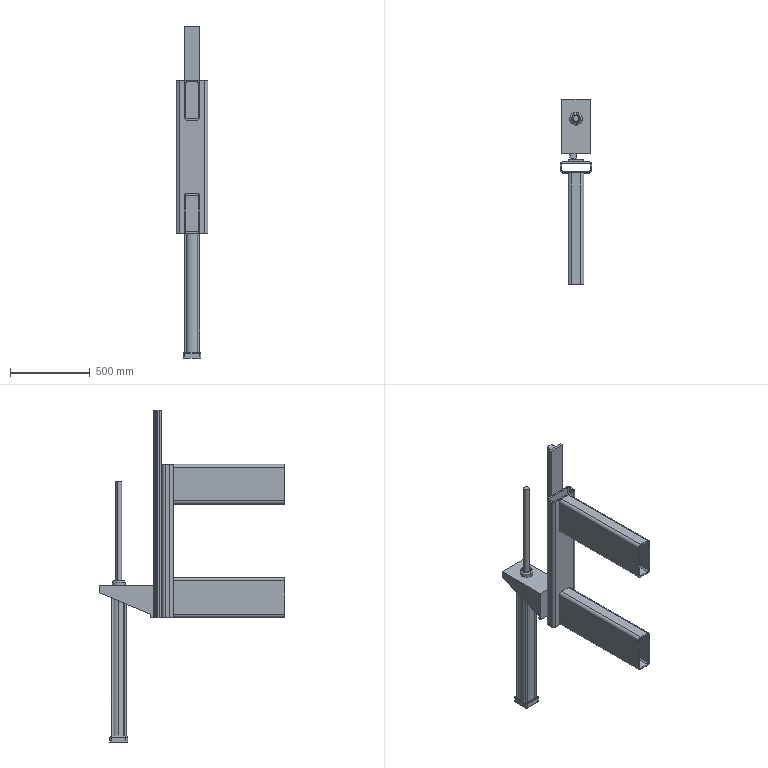Assembly | SolidWorks | mm | 15 component files | 15 solids | 255 faces | box 200 x 1164 x 2080 mm | volume 28088641 mm3 | cylinder 137 | plane 108 | torus 10 | commonest cylinder face diameters 30 x26 15.5 x26 15 x24 20 x20 40 x12 10 x11 85 x6 95 x4
Bill of materials:
CylinderBaseBaffle | 1 |  | Rectangular block with one sloped face. It is tall at one end and tapers to a thin end at the other. One round through-hole runs top to bottom, and a small step sits at the bottom of the tall end.
CylinderJoint | 1 | 1023 Carbon Steel Plate (SS) | Square flange base with rounded corners and edges, four corner through-holes, and a cylindrical boss in the middle. The boss has a rounded top edge and a central through-bore.
CylinderRod1 | 1 | 201 Annealed Stainless Steel (SS) | Solid round rod: a plain cylinder with flat ends.
CylinderWall1 | 1 | 201 Annealed Stainless Steel (SS) | Thin-walled round tube with open ends.
GuideRail2100 | 1 |  | Long, slender straight profile with a shaped cross-section and a row of evenly spaced small holes along one face.
GuideRailPad | 1 | Alloy Steel | Thin, flat rectangular strip or bar with no holes or other features.
MountingBracket | 1 | 1023 Carbon Steel Plate (SS) | Thick square plate with rounded corners and edges and four corner through-holes. One face has a large shallow circular recess.
Part10 | 2 | Electroplated Steel | Short length of thin-walled rectangular tube with rounded corners and open ends.
Part12 | 1 | Electroplated Steel | Thin-walled rectangular tube with rounded corners and open ends. It is longer and has a flatter cross-section than unnamed part.
PistonRod | 1 |  | Slender solid round rod: a plain cylinder with flat ends.
ScrewRod1 | 4 | 1023 Carbon Steel Plate (SS) | Very slender solid round rod or wire-like cylinder with flat ends.
Mates:
1. coincident | CylinderWall1-1 face at (-7.456, 2.584, -375) dir (0, 0, -1) | CylinderRod1-1 face at (-7.456, 2.584, -375) dir (0, 0, -1)
2. concentric | CylinderWall1-1 face at (-7.456, 2.584, 525) dir (0, 0, -1) r 47.5 | CylinderRod1-1 face at (-7.456, 2.584, 375) dir (0, 0, -1) r 42.5
3. coincident | CylinderWall1-1 face at (-7.456, 2.584, 525) dir (0, 0, 1) | CylinderJoint-1 face at (-62.456, -52.416, 525) dir (0, 0, -1)
4. concentric | CylinderWall1-1 face at (-7.456, 2.584, 525) dir (0, 0, -1) r 47.5 | CylinderJoint-1 face at (-7.456, 2.584, 610) dir (0, 0, -1) r 40
5. concentric | CylinderJoint-1 face at (-47.456, 42.584, 525) dir (0, 0, 1) r 7.5 | ScrewRod1-1 face at (-47.456, 42.584, 555.197) dir (0, 0, -1) r 7.5
6. coincident | CylinderRod1-1 face at (-7.456, 2.584, -375) dir (0, 0, -1) | MountingBracket-1 face at (-7.456, 2.584, -375) dir (0, 0, 1)
7. concentric | CylinderWall1-1 face at (-7.456, 2.584, 525) dir (0, 0, -1) r 47.5 | MountingBracket-1 face at (-7.456, 2.584, -375) dir (0, 0, 1) r 47.5
8. concentric | ScrewRod1-1 face at (-47.456, 42.584, 555.197) dir (0, 0, -1) r 7.5 | MountingBracket-1 face at (-47.456, 42.584, -400) dir (0, 0, 1) r 7.5
9. concentric | CylinderJoint-1 face at (32.544, 42.584, 525) dir (0, 0, 1) r 7.5 | ScrewRod1-2 face at (32.544, 42.584, 555.394) dir (0, 0, -1) r 7.5
10. concentric | MountingBracket-1 face at (32.544, 42.584, -400) dir (0, 0, 1) r 7.5 | ScrewRod1-2 face at (32.544, 42.584, 555.394) dir (0, 0, -1) r 7.5
11. concentric | MountingBracket-1 edge at (-47.456, -37.416, -400) dir (0, 0, 1) r 7.5 | ScrewRod1-3 face at (-47.456, -37.416, 556.307) dir (0, 0, -1) r 7.5
12. concentric | MountingBracket-1 face at (32.544, -37.416, -400) dir (0, 0, 1) r 7.5 | ScrewRod1-4 face at (32.544, -37.416, 555.579) dir (0, 0, -1) r 7.5
13. concentric | CylinderWall1-1 face at (-7.456, 2.584, 525) dir (0, 0, -1) r 47.5 | PistonRod-1 face at (-7.456, 2.584, 1235) dir (0, 0, -1) r 17.5
14. coincident | CylinderJoint-1 face at (-62.456, -52.416, 560) dir (0, 0, 1) | CylinderBaseBaffle-1 face at (-97.456, 125.725, 560) dir (0, 0, -1)
15. parallel | CylinderJoint-1 face at (47.544, 57.584, 560) dir (0, 1, 0) | CylinderBaseBaffle-1 face at (-97.456, -194.275, 380) dir (0, 1, 0)
16. coincident | CylinderJoint-1 face at (-62.456, -52.416, 560) dir (0, 0, 1) | CylinderBaseBaffle-1 face at (-97.456, 125.725, 560) dir (0, 0, -1)
17. concentric | CylinderWall1-1 face at (-7.456, 2.584, 525) dir (0, 0, -1) r 47.5 | CylinderBaseBaffle-1 face at (-7.456, 2.584, 610) dir (0, 0, -1) r 40
18. coincident | CylinderBaseBaffle-1 face at (-97.456, -214.275, 380) dir (0, 0, -1) | Part12-1 face at (72.544, -318.275, 380) dir (0, 0, -1)
19. width | CylinderBaseBaffle-1 face at (82.544, -194.275, 580) dir (1, 0, 0) | CylinderBaseBaffle-1 face at (-97.456, -194.275, 580) dir (-1, 0, 0) | Part12-1 face at (-107.456, -318.275, 380) dir (-1, 0, 0) | Part12-1 face at (92.544, -318.275, 380) dir (1, 0, 0)
20. coincident | Part12-1 face at (-87.456, -338.275, 380) dir (0, -1, 0) | Part10-1 face at (-37.456, -338.275, 610) dir (0, 1, 0)
21. distance | Part12-1 face at (-107.456, -318.275, 380) dir (-1, 0, 0) | Part10-1 face at (-57.456, -1038.275, 400) dir (-1, 0, 0)
22. coincident | GuideRail2100-1 face at (-13.706, -252.275, 1680) dir (0, -1, 0) | GuideRailPad-1 face at (42.544, -252.275, 1680) dir (0, 1, 0)
23. coincident | Part12-1 face at (72.544, -318.275, 380) dir (0, 0, -1) | Part10-1 face at (-37.456, -1038.275, 380) dir (0, 0, -1)
24. coincident | Part12-1 face at (-87.456, -338.275, 380) dir (0, -1, 0) | Part10-2 face at (-37.456, -338.275, 1320) dir (0, 1, 0)
25. coincident | Part10-1 face at (-57.456, -1038.275, 400) dir (-1, 0, 0) | Part10-2 face at (-57.456, -1038.275, 1110) dir (-1, 0, 0)
26. coincident | Part12-1 face at (72.544, -318.275, 1340) dir (0, 0, 1) | Part10-2 face at (-37.456, -1038.275, 1340) dir (0, 0, 1)
27. coincident | Part12-1 face at (-87.456, -268.275, 380) dir (0, 1, 0) | GuideRailPad-1 face at (42.544, -268.275, 1680) dir (0, -1, 0)
28. coincident | Part12-1 face at (72.544, -318.275, 380) dir (0, 0, -1) | GuideRailPad-1 face at (-57.456, -252.275, 380) dir (0, 0, -1)
29. coincident | GuideRailPad-1 face at (-57.456, -252.275, 380) dir (0, 0, -1) | GuideRail2100-1 face at (-1.206, -215.404, 380) dir (0, 0, -1)
30. coincident | CylinderBaseBaffle-1 face at (-97.456, -214.275, 380) dir (0, -1, 0) | GuideRail2100-1 face at (-41.335, -214.275, 1680) dir (0, 1, 0)
31. coincident | CylinderRod1-1 face at (-7.456, 2.584, 375) dir (0, 0, 1) | PistonRod-1 face at (-7.456, 2.584, 375) dir (0, 0, -1)